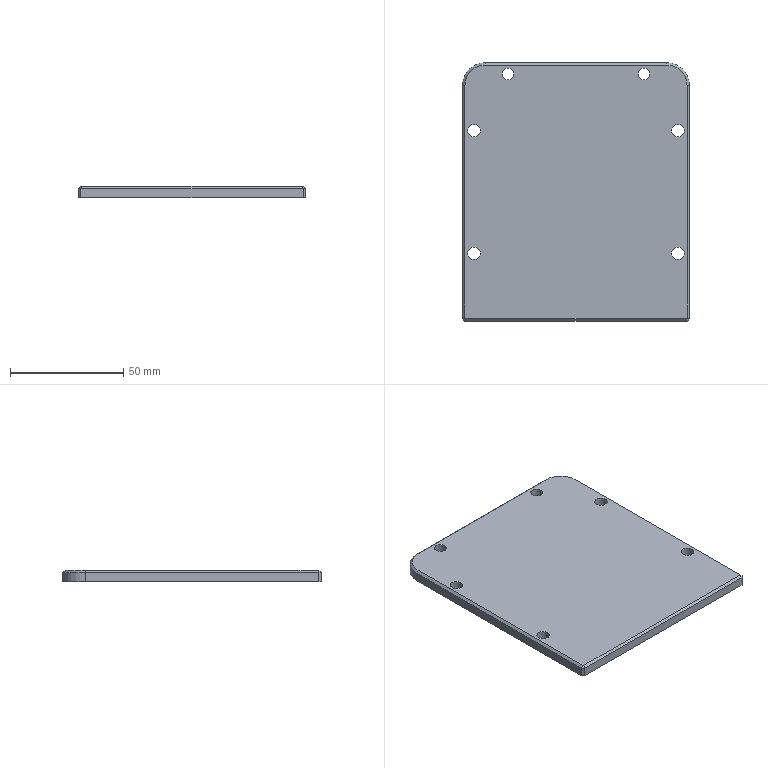CAM job | Mastercam | mm | 7 operations | part box 100 x 114 x 5
1. Facing | 12 - 12 平铣刀
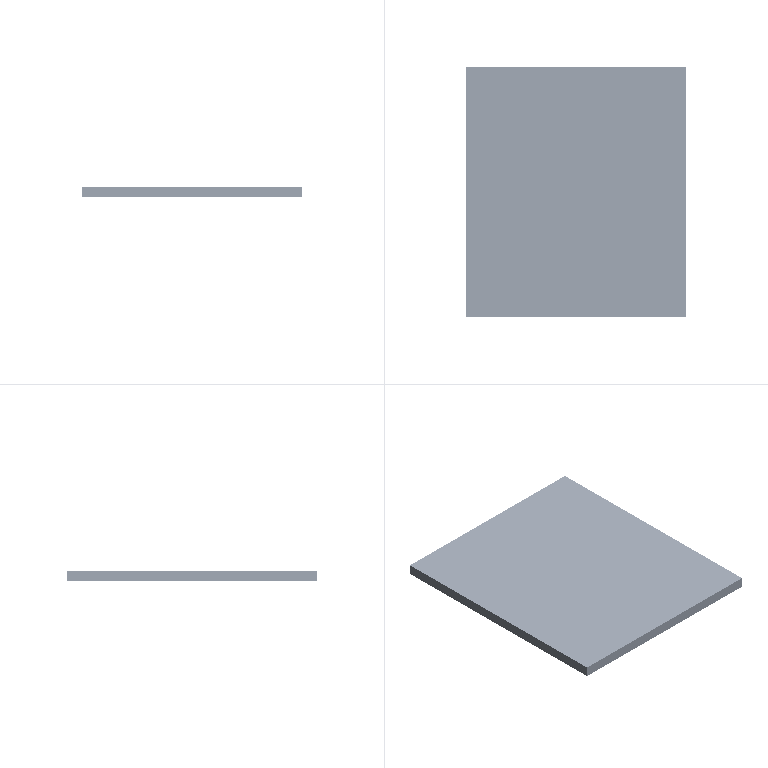2. Contour (Ramp) | 12 - 12 平铣刀
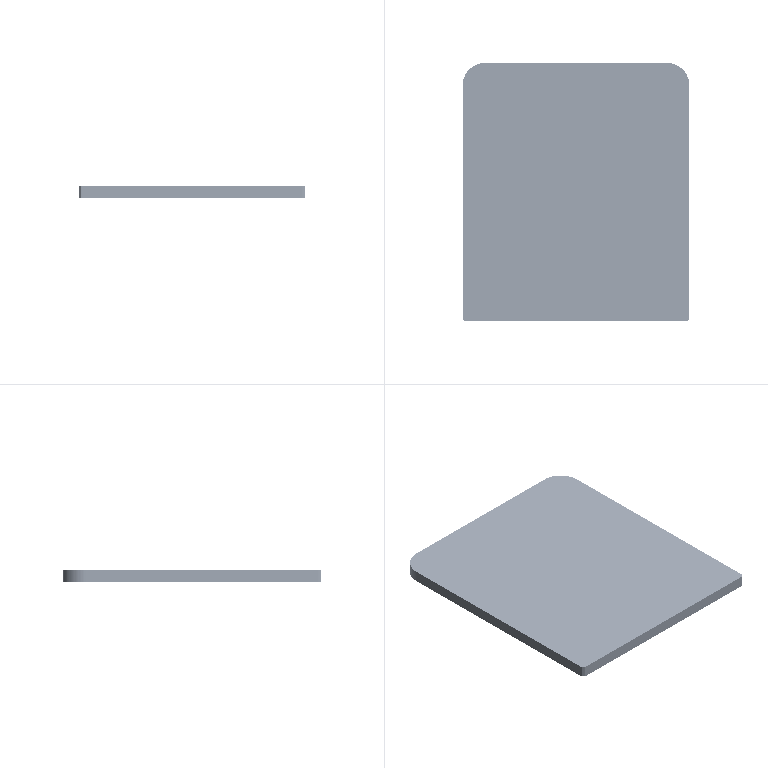3. Contour (2D) | 12 - 12 平铣刀
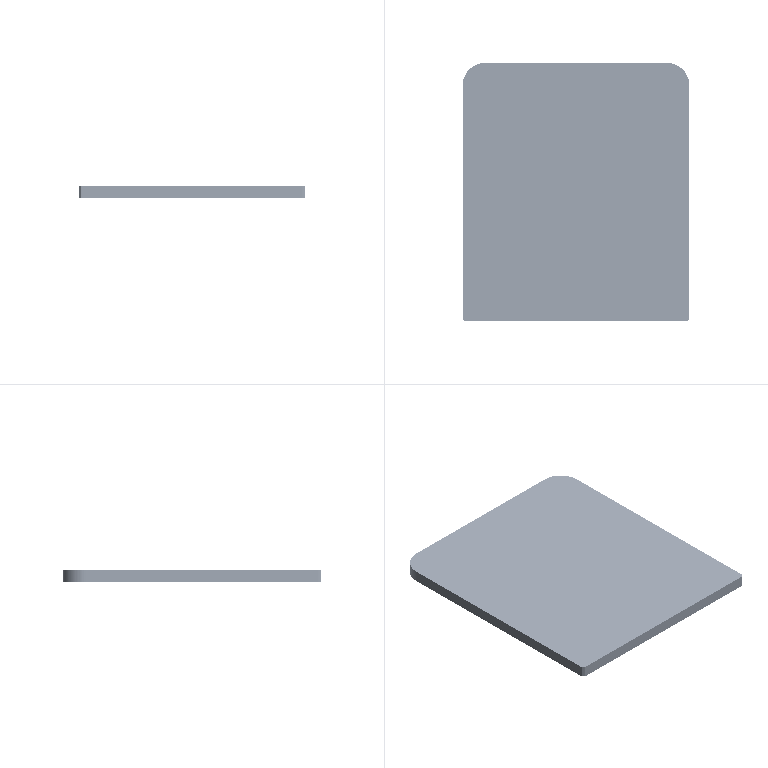4. Contour (2D chamfer) | 7 - 4 倒角刀
5. Drill/Counterbore | 7 - 4 倒角刀
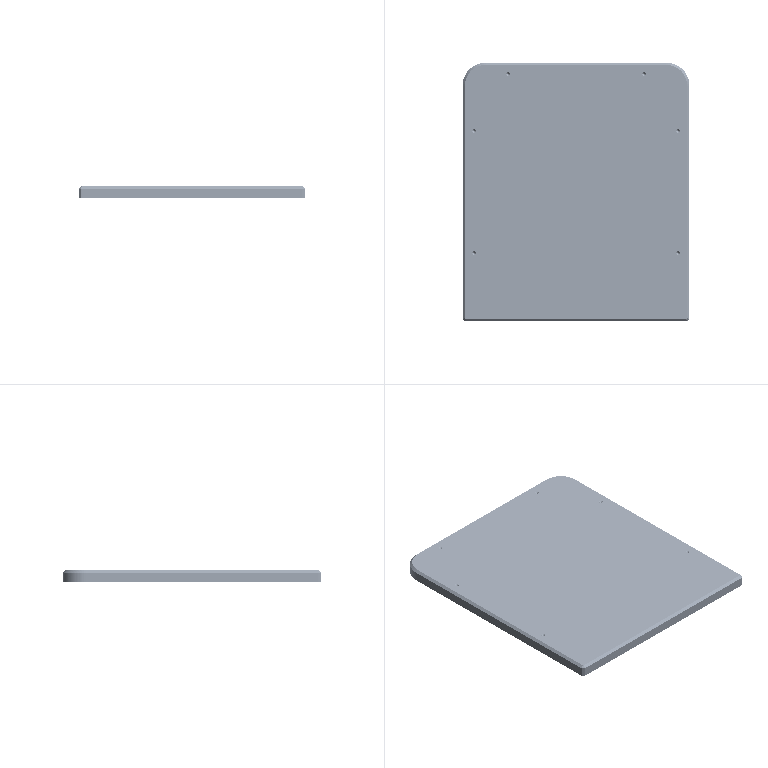6. Facing | 12 - 12 平铣刀
7. Contour (2D chamfer) | 7 - 4 倒角刀